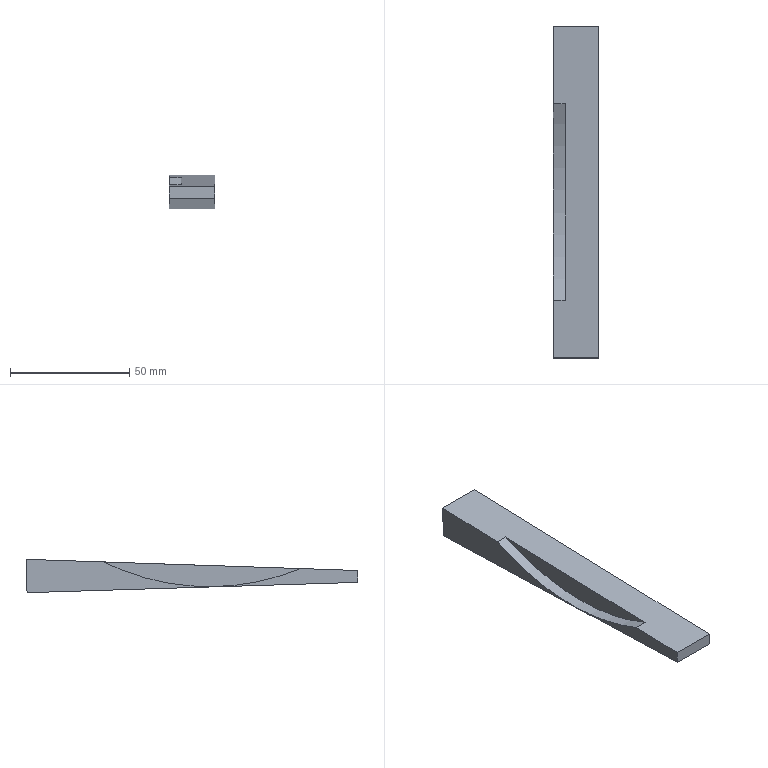Component | NX | LOWER_WEDGE | 1 solid | 8 faces | box 19 x 139.37 x 13.99 mm | volume 22605 mm3 | plane 7 | cylinder 1 | commonest cylinder face diameters 200.185 x1
STEP:
#1=CARTESIAN_POINT('',(0.,0.,0.));
#2=DIRECTION('',(0.,0.,1.));
#3=DIRECTION('',(1.,0.,0.));
#4=AXIS2_PLACEMENT_3D('',#1,#2,#3);
#5=CARTESIAN_POINT('',(-95.,83.,62.429));
#6=VERTEX_POINT('',#5);
#7=CARTESIAN_POINT('',(-95.,82.565,48.436));
#8=VERTEX_POINT('',#7);
#9=CARTESIAN_POINT('',(-95.,83.,62.429));
#10=DIRECTION('',(0.,-0.03104,-0.9995));
#11=VECTOR('',#10,1.);
#12=LINE('',#9,#11);
#13=CARTESIAN_POINT('',(-114.,83.,62.429));
#14=DIRECTION('',(0.,-0.9995,0.03104));
#15=DIRECTION('',(0.,0.03104,0.9995));
#16=AXIS2_PLACEMENT_3D('',#13,#14,#15);
#17=PLANE('',#16);
#18=CARTESIAN_POINT('',(0.,-19.));
#19=DIRECTION('',(-1.,0.));
#20=VECTOR('',#19,1.);
#21=LINE('',#18,#20);
#22=(GEOMETRIC_REPRESENTATION_CONTEXT(2)PARAMETRIC_REPRESENTATION_CONTEXT()REPRESENTATION_CONTEXT('',''));
#23=DEFINITIONAL_REPRESENTATION('',(#21),#22);
#24=PCURVE('',#17,#23);
#25=CARTESIAN_POINT('',(-95.,83.,62.429));
#26=DIRECTION('',(-1.,0.,0.));
#27=DIRECTION('',(0.,-0.03104,-0.9995));
#28=AXIS2_PLACEMENT_3D('',#25,#26,#27);
#29=PLANE('',#28);
#30=CARTESIAN_POINT('',(0.,0.));
#31=DIRECTION('',(1.,-0.));
#32=VECTOR('',#31,1.);
#33=LINE('',#30,#32);
#34=(GEOMETRIC_REPRESENTATION_CONTEXT(2)PARAMETRIC_REPRESENTATION_CONTEXT()REPRESENTATION_CONTEXT('',''));
#35=DEFINITIONAL_REPRESENTATION('',(#33),#34);
#36=PCURVE('',#29,#35);
#37=SURFACE_CURVE('',#12,(#24,#36),.PCURVE_S1.);
#38=EDGE_CURVE('',#6,#8,#37,.T.);
#39=ORIENTED_EDGE('',*,*,#38,.T.);
#40=CARTESIAN_POINT('',(-114.,82.565,48.436));
#41=VERTEX_POINT('',#40);
#42=CARTESIAN_POINT('',(-114.,82.565,48.436));
#43=DIRECTION('',(1.,0.,0.));
#44=VECTOR('',#43,1.);
#45=LINE('',#42,#44);
#46=CARTESIAN_POINT('',(-14.,0.));
#47=DIRECTION('',(0.,-1.));
#48=VECTOR('',#47,1.);
#49=LINE('',#46,#48);
#50=(GEOMETRIC_REPRESENTATION_CONTEXT(2)PARAMETRIC_REPRESENTATION_CONTEXT()REPRESENTATION_CONTEXT('',''));
#51=DEFINITIONAL_REPRESENTATION('',(#49),#50);
#52=PCURVE('',#17,#51);
#53=CARTESIAN_POINT('',(-114.,82.565,48.436));
#54=DIRECTION('',(0.,0.03104,0.9995));
#55=DIRECTION('',(0.,0.9995,-0.03104));
#56=AXIS2_PLACEMENT_3D('',#53,#54,#55);
#57=PLANE('',#56);
#58=CARTESIAN_POINT('',(0.,0.));
#59=DIRECTION('',(0.,-1.));
#60=VECTOR('',#59,1.);
#61=LINE('',#58,#60);
#62=(GEOMETRIC_REPRESENTATION_CONTEXT(2)PARAMETRIC_REPRESENTATION_CONTEXT()REPRESENTATION_CONTEXT('',''));
#63=DEFINITIONAL_REPRESENTATION('',(#61),#62);
#64=PCURVE('',#57,#63);
#65=SURFACE_CURVE('',#45,(#52,#64),.PCURVE_S1.);
#66=EDGE_CURVE('',#41,#8,#65,.T.);
#67=ORIENTED_EDGE('',*,*,#66,.F.);
#68=CARTESIAN_POINT('',(-114.,83.,62.429));
#69=VERTEX_POINT('',#68);
#70=CARTESIAN_POINT('',(-114.,83.,62.429));
#71=DIRECTION('',(0.,-0.03104,-0.9995));
#72=VECTOR('',#71,1.);
#73=LINE('',#70,#72);
#74=CARTESIAN_POINT('',(0.,0.));
#75=DIRECTION('',(-1.,0.));
#76=VECTOR('',#75,1.);
#77=LINE('',#74,#76);
#78=(GEOMETRIC_REPRESENTATION_CONTEXT(2)PARAMETRIC_REPRESENTATION_CONTEXT()REPRESENTATION_CONTEXT('',''));
#79=DEFINITIONAL_REPRESENTATION('',(#77),#78);
#80=PCURVE('',#17,#79);
#81=CARTESIAN_POINT('',(-114.,83.,62.429));
#82=DIRECTION('',(-1.,0.,0.));
#83=DIRECTION('',(0.,-0.03104,-0.9995));
#84=AXIS2_PLACEMENT_3D('',#81,#82,#83);
#85=PLANE('',#84);
#86=CARTESIAN_POINT('',(0.,0.));
#87=DIRECTION('',(1.,-0.));
#88=VECTOR('',#87,1.);
#89=LINE('',#86,#88);
#90=(GEOMETRIC_REPRESENTATION_CONTEXT(2)PARAMETRIC_REPRESENTATION_CONTEXT()REPRESENTATION_CONTEXT('',''));
#91=DEFINITIONAL_REPRESENTATION('',(#89),#90);
#92=PCURVE('',#85,#91);
#93=SURFACE_CURVE('',#73,(#80,#92),.PCURVE_S1.);
#94=EDGE_CURVE('',#69,#41,#93,.T.);
#95=ORIENTED_EDGE('',*,*,#94,.F.);
#96=CARTESIAN_POINT('',(-114.,83.,62.429));
#97=DIRECTION('',(1.,0.,0.));
#98=VECTOR('',#97,1.);
#99=LINE('',#96,#98);
#100=CARTESIAN_POINT('',(0.,0.));
#101=DIRECTION('',(0.,-1.));
#102=VECTOR('',#101,1.);
#103=LINE('',#100,#102);
#104=(GEOMETRIC_REPRESENTATION_CONTEXT(2)PARAMETRIC_REPRESENTATION_CONTEXT()REPRESENTATION_CONTEXT('',''));
#105=DEFINITIONAL_REPRESENTATION('',(#103),#104);
#106=PCURVE('',#17,#105);
#107=CARTESIAN_POINT('',(-114.,-56.212,57.748));
#108=DIRECTION('',(0.,0.03361,-0.9994));
#109=DIRECTION('',(0.,-0.9994,-0.03361));
#110=AXIS2_PLACEMENT_3D('',#107,#108,#109);
#111=PLANE('',#110);
#112=CARTESIAN_POINT('',(-139.291,0.));
#113=DIRECTION('',(0.,-1.));
#114=VECTOR('',#113,1.);
#115=LINE('',#112,#114);
#116=(GEOMETRIC_REPRESENTATION_CONTEXT(2)PARAMETRIC_REPRESENTATION_CONTEXT()REPRESENTATION_CONTEXT('',''));
#117=DEFINITIONAL_REPRESENTATION('',(#115),#116);
#118=PCURVE('',#111,#117);
#119=SURFACE_CURVE('',#99,(#106,#118),.PCURVE_S1.);
#120=EDGE_CURVE('',#69,#6,#119,.T.);
#121=ORIENTED_EDGE('',*,*,#120,.T.);
#122=EDGE_LOOP('',(#39,#67,#95,#121));
#123=FACE_BOUND('',#122,.T.);
#124=ADVANCED_FACE('',(#123),#17,.F.);
#125=CARTESIAN_POINT('',(-95.,-56.368,52.751));
#126=VERTEX_POINT('',#125);
#127=CARTESIAN_POINT('',(-95.,82.565,48.436));
#128=DIRECTION('',(0.,-0.9995,0.03104));
#129=VECTOR('',#128,1.);
#130=LINE('',#127,#129);
#131=CARTESIAN_POINT('',(0.,-19.));
#132=DIRECTION('',(-1.,0.));
#133=VECTOR('',#132,1.);
#134=LINE('',#131,#133);
#135=(GEOMETRIC_REPRESENTATION_CONTEXT(2)PARAMETRIC_REPRESENTATION_CONTEXT()REPRESENTATION_CONTEXT('',''));
#136=DEFINITIONAL_REPRESENTATION('',(#134),#135);
#137=PCURVE('',#57,#136);
#138=CARTESIAN_POINT('',(14.,-0.));
#139=DIRECTION('',(-0.,1.));
#140=VECTOR('',#139,1.);
#141=LINE('',#138,#140);
#142=(GEOMETRIC_REPRESENTATION_CONTEXT(2)PARAMETRIC_REPRESENTATION_CONTEXT()REPRESENTATION_CONTEXT('',''));
#143=DEFINITIONAL_REPRESENTATION('',(#141),#142);
#144=PCURVE('',#29,#143);
#145=SURFACE_CURVE('',#130,(#137,#144),.PCURVE_S1.);
#146=EDGE_CURVE('',#8,#126,#145,.T.);
#147=ORIENTED_EDGE('',*,*,#146,.T.);
#148=CARTESIAN_POINT('',(-114.,-56.368,52.751));
#149=VERTEX_POINT('',#148);
#150=CARTESIAN_POINT('',(-114.,-56.368,52.751));
#151=DIRECTION('',(1.,0.,0.));
#152=VECTOR('',#151,1.);
#153=LINE('',#150,#152);
#154=CARTESIAN_POINT('',(-139.,0.));
#155=DIRECTION('',(0.,-1.));
#156=VECTOR('',#155,1.);
#157=LINE('',#154,#156);
#158=(GEOMETRIC_REPRESENTATION_CONTEXT(2)PARAMETRIC_REPRESENTATION_CONTEXT()REPRESENTATION_CONTEXT('',''));
#159=DEFINITIONAL_REPRESENTATION('',(#157),#158);
#160=PCURVE('',#57,#159);
#161=CARTESIAN_POINT('',(-114.,-56.368,52.751));
#162=DIRECTION('',(0.,0.9995,-0.03104));
#163=DIRECTION('',(0.,-0.03104,-0.9995));
#164=AXIS2_PLACEMENT_3D('',#161,#162,#163);
#165=PLANE('',#164);
#166=CARTESIAN_POINT('',(0.,0.));
#167=DIRECTION('',(0.,-1.));
#168=VECTOR('',#167,1.);
#169=LINE('',#166,#168);
#170=(GEOMETRIC_REPRESENTATION_CONTEXT(2)PARAMETRIC_REPRESENTATION_CONTEXT()REPRESENTATION_CONTEXT('',''));
#171=DEFINITIONAL_REPRESENTATION('',(#169),#170);
#172=PCURVE('',#165,#171);
#173=SURFACE_CURVE('',#153,(#160,#172),.PCURVE_S1.);
#174=EDGE_CURVE('',#149,#126,#173,.T.);
#175=ORIENTED_EDGE('',*,*,#174,.F.);
#176=CARTESIAN_POINT('',(-114.,82.565,48.436));
#177=DIRECTION('',(0.,-0.9995,0.03104));
#178=VECTOR('',#177,1.);
#179=LINE('',#176,#178);
#180=CARTESIAN_POINT('',(0.,0.));
#181=DIRECTION('',(-1.,0.));
#182=VECTOR('',#181,1.);
#183=LINE('',#180,#182);
#184=(GEOMETRIC_REPRESENTATION_CONTEXT(2)PARAMETRIC_REPRESENTATION_CONTEXT()REPRESENTATION_CONTEXT('',''));
#185=DEFINITIONAL_REPRESENTATION('',(#183),#184);
#186=PCURVE('',#57,#185);
#187=CARTESIAN_POINT('',(14.,-0.));
#188=DIRECTION('',(-0.,1.));
#189=VECTOR('',#188,1.);
#190=LINE('',#187,#189);
#191=(GEOMETRIC_REPRESENTATION_CONTEXT(2)PARAMETRIC_REPRESENTATION_CONTEXT()REPRESENTATION_CONTEXT('',''));
#192=DEFINITIONAL_REPRESENTATION('',(#190),#191);
#193=PCURVE('',#85,#192);
#194=SURFACE_CURVE('',#179,(#186,#193),.PCURVE_S1.);
#195=EDGE_CURVE('',#41,#149,#194,.T.);
#196=ORIENTED_EDGE('',*,*,#195,.F.);
#197=ORIENTED_EDGE('',*,*,#66,.T.);
#198=EDGE_LOOP('',(#147,#175,#196,#197));
#199=FACE_BOUND('',#198,.T.);
#200=ADVANCED_FACE('',(#199),#57,.F.);
#201=CARTESIAN_POINT('',(-95.,-56.212,57.748));
#202=VERTEX_POINT('',#201);
#203=CARTESIAN_POINT('',(-95.,-56.368,52.751));
#204=DIRECTION('',(0.,0.03104,0.9995));
#205=VECTOR('',#204,1.);
#206=LINE('',#203,#205);
#207=CARTESIAN_POINT('',(0.,-19.));
#208=DIRECTION('',(-1.,0.));
#209=VECTOR('',#208,1.);
#210=LINE('',#207,#209);
#211=(GEOMETRIC_REPRESENTATION_CONTEXT(2)PARAMETRIC_REPRESENTATION_CONTEXT()REPRESENTATION_CONTEXT('',''));
#212=DEFINITIONAL_REPRESENTATION('',(#210),#211);
#213=PCURVE('',#165,#212);
#214=CARTESIAN_POINT('',(14.,139.));
#215=DIRECTION('',(-1.,0.));
#216=VECTOR('',#215,1.);
#217=LINE('',#214,#216);
#218=(GEOMETRIC_REPRESENTATION_CONTEXT(2)PARAMETRIC_REPRESENTATION_CONTEXT()REPRESENTATION_CONTEXT('',''));
#219=DEFINITIONAL_REPRESENTATION('',(#217),#218);
#220=PCURVE('',#29,#219);
#221=SURFACE_CURVE('',#206,(#213,#220),.PCURVE_S1.);
#222=EDGE_CURVE('',#126,#202,#221,.T.);
#223=ORIENTED_EDGE('',*,*,#222,.T.);
#224=CARTESIAN_POINT('',(-114.,-56.212,57.748));
#225=VERTEX_POINT('',#224);
#226=CARTESIAN_POINT('',(-114.,-56.212,57.748));
#227=DIRECTION('',(1.,0.,0.));
#228=VECTOR('',#227,1.);
#229=LINE('',#226,#228);
#230=CARTESIAN_POINT('',(-5.,0.));
#231=DIRECTION('',(0.,-1.));
#232=VECTOR('',#231,1.);
#233=LINE('',#230,#232);
#234=(GEOMETRIC_REPRESENTATION_CONTEXT(2)PARAMETRIC_REPRESENTATION_CONTEXT()REPRESENTATION_CONTEXT('',''));
#235=DEFINITIONAL_REPRESENTATION('',(#233),#234);
#236=PCURVE('',#165,#235);
#237=CARTESIAN_POINT('',(0.,0.));
#238=DIRECTION('',(0.,-1.));
#239=VECTOR('',#238,1.);
#240=LINE('',#237,#239);
#241=(GEOMETRIC_REPRESENTATION_CONTEXT(2)PARAMETRIC_REPRESENTATION_CONTEXT()REPRESENTATION_CONTEXT('',''));
#242=DEFINITIONAL_REPRESENTATION('',(#240),#241);
#243=PCURVE('',#111,#242);
#244=SURFACE_CURVE('',#229,(#236,#243),.PCURVE_S1.);
#245=EDGE_CURVE('',#225,#202,#244,.T.);
#246=ORIENTED_EDGE('',*,*,#245,.F.);
#247=CARTESIAN_POINT('',(-114.,-56.368,52.751));
#248=DIRECTION('',(0.,0.03104,0.9995));
#249=VECTOR('',#248,1.);
#250=LINE('',#247,#249);
#251=CARTESIAN_POINT('',(0.,0.));
#252=DIRECTION('',(-1.,0.));
#253=VECTOR('',#252,1.);
#254=LINE('',#251,#253);
#255=(GEOMETRIC_REPRESENTATION_CONTEXT(2)PARAMETRIC_REPRESENTATION_CONTEXT()REPRESENTATION_CONTEXT('',''));
#256=DEFINITIONAL_REPRESENTATION('',(#254),#255);
#257=PCURVE('',#165,#256);
#258=CARTESIAN_POINT('',(14.,139.));
#259=DIRECTION('',(-1.,0.));
#260=VECTOR('',#259,1.);
#261=LINE('',#258,#260);
#262=(GEOMETRIC_REPRESENTATION_CONTEXT(2)PARAMETRIC_REPRESENTATION_CONTEXT()REPRESENTATION_CONTEXT('',''));
#263=DEFINITIONAL_REPRESENTATION('',(#261),#262);
#264=PCURVE('',#85,#263);
#265=SURFACE_CURVE('',#250,(#257,#264),.PCURVE_S1.);
#266=EDGE_CURVE('',#149,#225,#265,.T.);
#267=ORIENTED_EDGE('',*,*,#266,.F.);
#268=ORIENTED_EDGE('',*,*,#174,.T.);
#269=EDGE_LOOP('',(#223,#246,#267,#268));
#270=FACE_BOUND('',#269,.T.);
#271=ADVANCED_FACE('',(#270),#165,.F.);
#272=CARTESIAN_POINT('',(-109.,-32.176,58.556));
#273=VERTEX_POINT('',#272);
#274=CARTESIAN_POINT('',(-109.,50.45,61.335));
#275=VERTEX_POINT('',#274);
#276=CARTESIAN_POINT('',(-109.,-32.176,58.556));
#277=DIRECTION('',(0.,0.9994,0.03361));
#278=VECTOR('',#277,1.);
#279=LINE('',#276,#278);
#280=CARTESIAN_POINT('',(-24.05,-5.));
#281=DIRECTION('',(-1.,0.));
#282=VECTOR('',#281,1.);
#283=LINE('',#280,#282);
#284=(GEOMETRIC_REPRESENTATION_CONTEXT(2)PARAMETRIC_REPRESENTATION_CONTEXT()REPRESENTATION_CONTEXT('',''));
#285=DEFINITIONAL_REPRESENTATION('',(#283),#284);
#286=PCURVE('',#111,#285);
#287=CARTESIAN_POINT('',(-109.,6.074,151.052));
#288=DIRECTION('',(-1.,0.,0.));
#289=DIRECTION('',(0.,-0.03104,-0.9995));
#290=AXIS2_PLACEMENT_3D('',#287,#288,#289);
#291=PLANE('',#290);
#292=CARTESIAN_POINT('',(93.638,35.36));
#293=DIRECTION('',(-0.06461,-0.9979));
#294=VECTOR('',#293,1.);
#295=LINE('',#292,#294);
#296=(GEOMETRIC_REPRESENTATION_CONTEXT(2)PARAMETRIC_REPRESENTATION_CONTEXT()REPRESENTATION_CONTEXT('',''));
#297=DEFINITIONAL_REPRESENTATION('',(#295),#296);
#298=PCURVE('',#291,#297);
#299=SURFACE_CURVE('',#279,(#286,#298),.PCURVE_S1.);
#300=EDGE_CURVE('',#273,#275,#299,.T.);
#301=ORIENTED_EDGE('',*,*,#300,.F.);
#302=CARTESIAN_POINT('',(-114.,-32.176,58.556));
#303=VERTEX_POINT('',#302);
#304=CARTESIAN_POINT('',(-109.,-32.176,58.556));
#305=DIRECTION('',(-1.,0.,0.));
#306=VECTOR('',#305,1.);
#307=LINE('',#304,#306);
#308=CARTESIAN_POINT('',(-24.05,-5.));
#309=DIRECTION('',(0.,1.));
#310=VECTOR('',#309,1.);
#311=LINE('',#308,#310);
#312=(GEOMETRIC_REPRESENTATION_CONTEXT(2)PARAMETRIC_REPRESENTATION_CONTEXT()REPRESENTATION_CONTEXT('',''));
#313=DEFINITIONAL_REPRESENTATION('',(#311),#312);
#314=PCURVE('',#111,#313);
#315=CARTESIAN_POINT('',(-109.,6.074,151.052));
#316=DIRECTION('',(-1.,0.,0.));
#317=DIRECTION('',(0.,-0.03104,-0.9995));
#318=AXIS2_PLACEMENT_3D('',#315,#316,#317);
#319=CYLINDRICAL_SURFACE('',#318,100.092);
#320=CARTESIAN_POINT('',(6.644,0.));
#321=DIRECTION('',(0.,1.));
#322=VECTOR('',#321,1.);
#323=LINE('',#320,#322);
#324=(GEOMETRIC_REPRESENTATION_CONTEXT(2)PARAMETRIC_REPRESENTATION_CONTEXT()REPRESENTATION_CONTEXT('',''));
#325=DEFINITIONAL_REPRESENTATION('',(#323),#324);
#326=PCURVE('',#319,#325);
#327=SURFACE_CURVE('',#307,(#314,#326),.PCURVE_S1.);
#328=EDGE_CURVE('',#273,#303,#327,.T.);
#329=ORIENTED_EDGE('',*,*,#328,.T.);
#330=CARTESIAN_POINT('',(-114.,-56.212,57.748));
#331=DIRECTION('',(0.,0.9994,0.03361));
#332=VECTOR('',#331,1.);
#333=LINE('',#330,#332);
#334=CARTESIAN_POINT('',(0.,0.));
#335=DIRECTION('',(-1.,0.));
#336=VECTOR('',#335,1.);
#337=LINE('',#334,#336);
#338=(GEOMETRIC_REPRESENTATION_CONTEXT(2)PARAMETRIC_REPRESENTATION_CONTEXT()REPRESENTATION_CONTEXT('',''));
#339=DEFINITIONAL_REPRESENTATION('',(#337),#338);
#340=PCURVE('',#111,#339);
#341=CARTESIAN_POINT('',(9.,139.));
#342=DIRECTION('',(-0.06461,-0.9979));
#343=VECTOR('',#342,1.);
#344=LINE('',#341,#343);
#345=(GEOMETRIC_REPRESENTATION_CONTEXT(2)PARAMETRIC_REPRESENTATION_CONTEXT()REPRESENTATION_CONTEXT('',''));
#346=DEFINITIONAL_REPRESENTATION('',(#344),#345);
#347=PCURVE('',#85,#346);
#348=SURFACE_CURVE('',#333,(#340,#347),.PCURVE_S1.);
#349=EDGE_CURVE('',#225,#303,#348,.T.);
#350=ORIENTED_EDGE('',*,*,#349,.F.);
#351=ORIENTED_EDGE('',*,*,#245,.T.);
#352=CARTESIAN_POINT('',(-95.,-56.212,57.748));
#353=DIRECTION('',(0.,0.9994,0.03361));
#354=VECTOR('',#353,1.);
#355=LINE('',#352,#354);
#356=CARTESIAN_POINT('',(0.,-19.));
#357=DIRECTION('',(-1.,0.));
#358=VECTOR('',#357,1.);
#359=LINE('',#356,#358);
#360=(GEOMETRIC_REPRESENTATION_CONTEXT(2)PARAMETRIC_REPRESENTATION_CONTEXT()REPRESENTATION_CONTEXT('',''));
#361=DEFINITIONAL_REPRESENTATION('',(#359),#360);
#362=PCURVE('',#111,#361);
#363=CARTESIAN_POINT('',(9.,139.));
#364=DIRECTION('',(-0.06461,-0.9979));
#365=VECTOR('',#364,1.);
#366=LINE('',#363,#365);
#367=(GEOMETRIC_REPRESENTATION_CONTEXT(2)PARAMETRIC_REPRESENTATION_CONTEXT()REPRESENTATION_CONTEXT('',''));
#368=DEFINITIONAL_REPRESENTATION('',(#366),#367);
#369=PCURVE('',#29,#368);
#370=SURFACE_CURVE('',#355,(#362,#369),.PCURVE_S1.);
#371=EDGE_CURVE('',#202,#6,#370,.T.);
#372=ORIENTED_EDGE('',*,*,#371,.T.);
#373=ORIENTED_EDGE('',*,*,#120,.F.);
#374=CARTESIAN_POINT('',(-114.,50.45,61.335));
#375=VERTEX_POINT('',#374);
#376=CARTESIAN_POINT('',(-114.,-56.212,57.748));
#377=DIRECTION('',(0.,0.9994,0.03361));
#378=VECTOR('',#377,1.);
#379=LINE('',#376,#378);
#380=CARTESIAN_POINT('',(0.,0.));
#381=DIRECTION('',(-1.,0.));
#382=VECTOR('',#381,1.);
#383=LINE('',#380,#382);
#384=(GEOMETRIC_REPRESENTATION_CONTEXT(2)PARAMETRIC_REPRESENTATION_CONTEXT()REPRESENTATION_CONTEXT('',''));
#385=DEFINITIONAL_REPRESENTATION('',(#383),#384);
#386=PCURVE('',#111,#385);
#387=CARTESIAN_POINT('',(9.,139.));
#388=DIRECTION('',(-0.06461,-0.9979));
#389=VECTOR('',#388,1.);
#390=LINE('',#387,#389);
#391=(GEOMETRIC_REPRESENTATION_CONTEXT(2)PARAMETRIC_REPRESENTATION_CONTEXT()REPRESENTATION_CONTEXT('',''));
#392=DEFINITIONAL_REPRESENTATION('',(#390),#391);
#393=PCURVE('',#85,#392);
#394=SURFACE_CURVE('',#379,(#386,#393),.PCURVE_S1.);
#395=EDGE_CURVE('',#375,#69,#394,.T.);
#396=ORIENTED_EDGE('',*,*,#395,.F.);
#397=CARTESIAN_POINT('',(-109.,50.45,61.335));
#398=DIRECTION('',(1.,0.,0.));
#399=VECTOR('',#398,1.);
#400=LINE('',#397,#399);
#401=CARTESIAN_POINT('',(-106.723,-5.));
#402=DIRECTION('',(0.,-1.));
#403=VECTOR('',#402,1.);
#404=LINE('',#401,#403);
#405=(GEOMETRIC_REPRESENTATION_CONTEXT(2)PARAMETRIC_REPRESENTATION_CONTEXT()REPRESENTATION_CONTEXT('',''));
#406=DEFINITIONAL_REPRESENTATION('',(#404),#405);
#407=PCURVE('',#111,#406);
#408=CARTESIAN_POINT('',(5.793,0.));
#409=DIRECTION('',(0.,-1.));
#410=VECTOR('',#409,1.);
#411=LINE('',#408,#410);
#412=(GEOMETRIC_REPRESENTATION_CONTEXT(2)PARAMETRIC_REPRESENTATION_CONTEXT()REPRESENTATION_CONTEXT('',''));
#413=DEFINITIONAL_REPRESENTATION('',(#411),#412);
#414=PCURVE('',#319,#413);
#415=SURFACE_CURVE('',#400,(#407,#414),.PCURVE_S1.);
#416=EDGE_CURVE('',#375,#275,#415,.T.);
#417=ORIENTED_EDGE('',*,*,#416,.T.);
#418=EDGE_LOOP('',(#301,#329,#350,#351,#372,#373,#396,#417));
#419=FACE_BOUND('',#418,.T.);
#420=ADVANCED_FACE('',(#419),#111,.F.);
#421=CARTESIAN_POINT('',(-114.,6.074,151.052));
#422=DIRECTION('',(-1.,0.,0.));
#423=DIRECTION('',(0.,-0.9995,0.03104));
#424=AXIS2_PLACEMENT_3D('',#421,#422,#423);
#425=CIRCLE('',#424,100.092);
#426=CARTESIAN_POINT('',(-86.192,79.64));
#427=DIRECTION('',(0.,1.));
#428=AXIS2_PLACEMENT_2D('',#426,#427);
#429=CIRCLE('',#428,100.092);
#430=(GEOMETRIC_REPRESENTATION_CONTEXT(2)PARAMETRIC_REPRESENTATION_CONTEXT()REPRESENTATION_CONTEXT('',''));
#431=DEFINITIONAL_REPRESENTATION('',(#429),#430);
#432=PCURVE('',#85,#431);
#433=CARTESIAN_POINT('',(1.571,5.));
#434=DIRECTION('',(1.,0.));
#435=VECTOR('',#434,1.);
#436=LINE('',#433,#435);
#437=(GEOMETRIC_REPRESENTATION_CONTEXT(2)PARAMETRIC_REPRESENTATION_CONTEXT()REPRESENTATION_CONTEXT('',''));
#438=DEFINITIONAL_REPRESENTATION('',(#436),#437);
#439=PCURVE('',#319,#438);
#440=SURFACE_CURVE('',#425,(#432,#439),.PCURVE_S1.);
#441=EDGE_CURVE('',#375,#303,#440,.T.);
#442=ORIENTED_EDGE('',*,*,#441,.F.);
#443=ORIENTED_EDGE('',*,*,#395,.T.);
#444=ORIENTED_EDGE('',*,*,#94,.T.);
#445=ORIENTED_EDGE('',*,*,#195,.T.);
#446=ORIENTED_EDGE('',*,*,#266,.T.);
#447=ORIENTED_EDGE('',*,*,#349,.T.);
#448=EDGE_LOOP('',(#442,#443,#444,#445,#446,#447));
#449=FACE_BOUND('',#448,.T.);
#450=ADVANCED_FACE('',(#449),#85,.T.);
#451=ORIENTED_EDGE('',*,*,#38,.F.);
#452=ORIENTED_EDGE('',*,*,#371,.F.);
#453=ORIENTED_EDGE('',*,*,#222,.F.);
#454=ORIENTED_EDGE('',*,*,#146,.F.);
#455=EDGE_LOOP('',(#451,#452,#453,#454));
#456=FACE_BOUND('',#455,.T.);
#457=ADVANCED_FACE('',(#456),#29,.F.);
#458=ORIENTED_EDGE('',*,*,#416,.T.);
#459=CARTESIAN_POINT('',(-109.,6.074,151.052));
#460=DIRECTION('',(1.,0.,0.));
#461=DIRECTION('',(0.,-0.9995,0.03104));
#462=AXIS2_PLACEMENT_3D('',#459,#460,#461);
#463=CIRCLE('',#462,100.092);
#464=CARTESIAN_POINT('',(7.854,0.));
#465=DIRECTION('',(-1.,0.));
#466=VECTOR('',#465,1.);
#467=LINE('',#464,#466);
#468=(GEOMETRIC_REPRESENTATION_CONTEXT(2)PARAMETRIC_REPRESENTATION_CONTEXT()REPRESENTATION_CONTEXT('',''));
#469=DEFINITIONAL_REPRESENTATION('',(#467),#468);
#470=PCURVE('',#319,#469);
#471=CARTESIAN_POINT('',(0.,100.092));
#472=CARTESIAN_POINT('',(173.365,100.092));
#473=CARTESIAN_POINT('',(86.683,-50.046));
#474=CARTESIAN_POINT('',(0.,-200.185));
#475=CARTESIAN_POINT('',(-86.683,-50.046));
#476=CARTESIAN_POINT('',(-173.365,100.092));
#477=CARTESIAN_POINT('',(0.,100.092));
#478=(BOUNDED_CURVE()B_SPLINE_CURVE(2,(#471,#472,#473,#474,#475,#476,#477),.UNSPECIFIED.,.T.,.F.)B_SPLINE_CURVE_WITH_KNOTS((1,2,2,2,2,1),(-2.094,0.,2.094,4.189,6.283,8.378),.UNSPECIFIED.)CURVE()GEOMETRIC_REPRESENTATION_ITEM()RATIONAL_B_SPLINE_CURVE((1.,0.5,1.,0.5,1.,0.5,1.))REPRESENTATION_ITEM(''));
#479=(GEOMETRIC_REPRESENTATION_CONTEXT(2)PARAMETRIC_REPRESENTATION_CONTEXT()REPRESENTATION_CONTEXT('',''));
#480=DEFINITIONAL_REPRESENTATION('',(#478),#479);
#481=PCURVE('',#291,#480);
#482=SURFACE_CURVE('',#463,(#470,#481),.PCURVE_S1.);
#483=EDGE_CURVE('',#273,#275,#482,.T.);
#484=ORIENTED_EDGE('',*,*,#483,.F.);
#485=ORIENTED_EDGE('',*,*,#328,.T.);
#486=ORIENTED_EDGE('',*,*,#441,.F.);
#487=EDGE_LOOP('',(#458,#484,#485,#486));
#488=FACE_BOUND('',#487,.F.);
#489=ADVANCED_FACE('',(#488),#319,.F.);
#490=ORIENTED_EDGE('',*,*,#483,.F.);
#491=ORIENTED_EDGE('',*,*,#300,.T.);
#492=EDGE_LOOP('',(#490,#491));
#493=FACE_BOUND('',#492,.T.);
#494=ADVANCED_FACE('',(#493),#291,.T.);
#495=CLOSED_SHELL('',(#124,#200,#271,#420,#450,#457,#489,#494));
#496=MANIFOLD_SOLID_BREP('',#495);
#497=(LENGTH_UNIT()NAMED_UNIT(*)SI_UNIT(.MILLI.,.METRE.));
#498=UNCERTAINTY_MEASURE_WITH_UNIT(LENGTH_MEASURE(0.0000001),#497,'','');
#499=(NAMED_UNIT(*)PLANE_ANGLE_UNIT()SI_UNIT($,.RADIAN.));
#500=(NAMED_UNIT(*)SI_UNIT($,.STERADIAN.)SOLID_ANGLE_UNIT());
#501=(GEOMETRIC_REPRESENTATION_CONTEXT(3)GLOBAL_UNCERTAINTY_ASSIGNED_CONTEXT((#498))GLOBAL_UNIT_ASSIGNED_CONTEXT((#497,#499,#500))REPRESENTATION_CONTEXT('',''));
#502=ADVANCED_BREP_SHAPE_REPRESENTATION('',(#4,#496),#501);